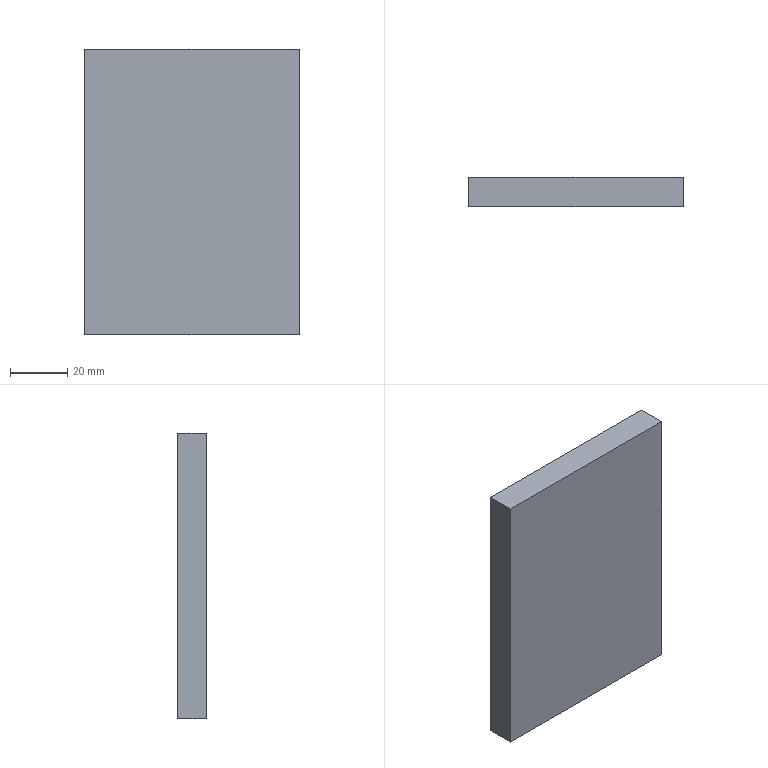Component | SolidWorks | TrolleyLeg-1_100X75X8-1 | 1 solid | 6 faces | box 75 x 10 x 100 mm | volume 75000 mm3 | plane 6 | material Plain Carbon Steel
STEP:
#1=COLOUR_RGB('',0.7922,0.8196,0.9333);
#2=FILL_AREA_STYLE_COLOUR('',#1);
#3=FILL_AREA_STYLE('',(#2));
#4=SURFACE_STYLE_FILL_AREA(#3);
#5=SURFACE_SIDE_STYLE('',(#4));
#6=SURFACE_STYLE_USAGE(.BOTH.,#5);
#7=PRESENTATION_STYLE_ASSIGNMENT((#6));
#8=CARTESIAN_POINT('',(-113.669,79.737,189.212));
#9=VERTEX_POINT('',#8);
#10=CARTESIAN_POINT('',(-113.669,79.737,185.275));
#11=VERTEX_POINT('',#10);
#12=CARTESIAN_POINT('',(-113.669,79.737,189.212));
#13=DIRECTION('',(0.,0.,-1.));
#14=VECTOR('',#13,39.37);
#15=LINE('',#12,#14);
#16=EDGE_CURVE('',#9,#11,#15,.T.);
#17=ORIENTED_EDGE('',*,*,#16,.F.);
#18=CARTESIAN_POINT('',(-113.669,80.131,189.212));
#19=VERTEX_POINT('',#18);
#20=CARTESIAN_POINT('',(-113.669,80.131,189.212));
#21=DIRECTION('',(0.,-1.,-0.));
#22=VECTOR('',#21,39.37);
#23=LINE('',#20,#22);
#24=EDGE_CURVE('',#19,#9,#23,.T.);
#25=ORIENTED_EDGE('',*,*,#24,.F.);
#26=CARTESIAN_POINT('',(-113.669,80.131,185.275));
#27=VERTEX_POINT('',#26);
#28=CARTESIAN_POINT('',(-113.669,80.131,189.212));
#29=DIRECTION('',(0.,0.,-1.));
#30=VECTOR('',#29,39.37);
#31=LINE('',#28,#30);
#32=EDGE_CURVE('',#19,#27,#31,.T.);
#33=ORIENTED_EDGE('',*,*,#32,.T.);
#34=CARTESIAN_POINT('',(-113.669,80.131,185.275));
#35=DIRECTION('',(0.,-1.,-0.));
#36=VECTOR('',#35,39.37);
#37=LINE('',#34,#36);
#38=EDGE_CURVE('',#27,#11,#37,.T.);
#39=ORIENTED_EDGE('',*,*,#38,.T.);
#40=EDGE_LOOP('',(#17,#25,#33,#39));
#41=FACE_OUTER_BOUND('',#40,.T.);
#42=CARTESIAN_POINT('',(-113.669,80.131,189.212));
#43=DIRECTION('',(-1.,0.,-0.));
#44=DIRECTION('',(0.,0.,-1.));
#45=AXIS2_PLACEMENT_3D('',#42,#43,#44);
#46=PLANE('',#45);
#47=ADVANCED_FACE('',(#41),#46,.T.);
#48=CARTESIAN_POINT('',(-110.717,79.737,189.212));
#49=VERTEX_POINT('',#48);
#50=CARTESIAN_POINT('',(-113.669,79.737,189.212));
#51=DIRECTION('',(-1.,0.,0.));
#52=VECTOR('',#51,39.37);
#53=LINE('',#50,#52);
#54=EDGE_CURVE('',#49,#9,#53,.T.);
#55=ORIENTED_EDGE('',*,*,#54,.F.);
#56=CARTESIAN_POINT('',(-110.717,80.131,189.212));
#57=VERTEX_POINT('',#56);
#58=CARTESIAN_POINT('',(-110.717,80.131,189.212));
#59=DIRECTION('',(0.,-1.,-0.));
#60=VECTOR('',#59,39.37);
#61=LINE('',#58,#60);
#62=EDGE_CURVE('',#57,#49,#61,.T.);
#63=ORIENTED_EDGE('',*,*,#62,.F.);
#64=CARTESIAN_POINT('',(-113.669,80.131,189.212));
#65=DIRECTION('',(-1.,0.,0.));
#66=VECTOR('',#65,39.37);
#67=LINE('',#64,#66);
#68=EDGE_CURVE('',#57,#19,#67,.T.);
#69=ORIENTED_EDGE('',*,*,#68,.T.);
#70=ORIENTED_EDGE('',*,*,#24,.T.);
#71=EDGE_LOOP('',(#55,#63,#69,#70));
#72=FACE_OUTER_BOUND('',#71,.T.);
#73=CARTESIAN_POINT('',(-113.669,80.131,189.212));
#74=DIRECTION('',(0.,-0.,1.));
#75=DIRECTION('',(-1.,0.,0.));
#76=AXIS2_PLACEMENT_3D('',#73,#74,#75);
#77=PLANE('',#76);
#78=ADVANCED_FACE('',(#72),#77,.T.);
#79=CARTESIAN_POINT('',(-110.717,79.737,185.275));
#80=VERTEX_POINT('',#79);
#81=CARTESIAN_POINT('',(-110.717,79.737,189.212));
#82=DIRECTION('',(-0.,-0.,1.));
#83=VECTOR('',#82,39.37);
#84=LINE('',#81,#83);
#85=EDGE_CURVE('',#80,#49,#84,.T.);
#86=ORIENTED_EDGE('',*,*,#85,.F.);
#87=CARTESIAN_POINT('',(-110.717,80.131,185.275));
#88=VERTEX_POINT('',#87);
#89=CARTESIAN_POINT('',(-110.717,80.131,185.275));
#90=DIRECTION('',(0.,-1.,-0.));
#91=VECTOR('',#90,39.37);
#92=LINE('',#89,#91);
#93=EDGE_CURVE('',#88,#80,#92,.T.);
#94=ORIENTED_EDGE('',*,*,#93,.F.);
#95=CARTESIAN_POINT('',(-110.717,80.131,189.212));
#96=DIRECTION('',(-0.,-0.,1.));
#97=VECTOR('',#96,39.37);
#98=LINE('',#95,#97);
#99=EDGE_CURVE('',#88,#57,#98,.T.);
#100=ORIENTED_EDGE('',*,*,#99,.T.);
#101=ORIENTED_EDGE('',*,*,#62,.T.);
#102=EDGE_LOOP('',(#86,#94,#100,#101));
#103=FACE_OUTER_BOUND('',#102,.T.);
#104=CARTESIAN_POINT('',(-110.717,80.131,189.212));
#105=DIRECTION('',(1.,-0.,0.));
#106=DIRECTION('',(-0.,-0.,1.));
#107=AXIS2_PLACEMENT_3D('',#104,#105,#106);
#108=PLANE('',#107);
#109=ADVANCED_FACE('',(#103),#108,.T.);
#110=CARTESIAN_POINT('',(-113.669,79.737,185.275));
#111=DIRECTION('',(1.,0.,0.));
#112=VECTOR('',#111,39.37);
#113=LINE('',#110,#112);
#114=EDGE_CURVE('',#11,#80,#113,.T.);
#115=ORIENTED_EDGE('',*,*,#114,.F.);
#116=ORIENTED_EDGE('',*,*,#38,.F.);
#117=CARTESIAN_POINT('',(-113.669,80.131,185.275));
#118=DIRECTION('',(1.,0.,0.));
#119=VECTOR('',#118,39.37);
#120=LINE('',#117,#119);
#121=EDGE_CURVE('',#27,#88,#120,.T.);
#122=ORIENTED_EDGE('',*,*,#121,.T.);
#123=ORIENTED_EDGE('',*,*,#93,.T.);
#124=EDGE_LOOP('',(#115,#116,#122,#123));
#125=FACE_OUTER_BOUND('',#124,.T.);
#126=CARTESIAN_POINT('',(-113.669,80.131,185.275));
#127=DIRECTION('',(0.,0.,-1.));
#128=DIRECTION('',(1.,0.,0.));
#129=AXIS2_PLACEMENT_3D('',#126,#127,#128);
#130=PLANE('',#129);
#131=ADVANCED_FACE('',(#125),#130,.T.);
#132=ORIENTED_EDGE('',*,*,#32,.F.);
#133=ORIENTED_EDGE('',*,*,#68,.F.);
#134=ORIENTED_EDGE('',*,*,#99,.F.);
#135=ORIENTED_EDGE('',*,*,#121,.F.);
#136=EDGE_LOOP('',(#132,#133,#134,#135));
#137=FACE_OUTER_BOUND('',#136,.T.);
#138=CARTESIAN_POINT('',(-113.669,80.131,189.212));
#139=DIRECTION('',(0.,-1.,-0.));
#140=DIRECTION('',(0.,0.,-1.));
#141=AXIS2_PLACEMENT_3D('',#138,#139,#140);
#142=PLANE('',#141);
#143=ADVANCED_FACE('',(#137),#142,.F.);
#144=ORIENTED_EDGE('',*,*,#16,.T.);
#145=ORIENTED_EDGE('',*,*,#114,.T.);
#146=ORIENTED_EDGE('',*,*,#85,.T.);
#147=ORIENTED_EDGE('',*,*,#54,.T.);
#148=EDGE_LOOP('',(#144,#145,#146,#147));
#149=FACE_OUTER_BOUND('',#148,.T.);
#150=CARTESIAN_POINT('',(-113.669,79.737,189.212));
#151=DIRECTION('',(0.,-1.,-0.));
#152=DIRECTION('',(0.,0.,-1.));
#153=AXIS2_PLACEMENT_3D('',#150,#151,#152);
#154=PLANE('',#153);
#155=ADVANCED_FACE('',(#149),#154,.T.);
#156=CLOSED_SHELL('',(#47,#78,#109,#131,#143,#155));
#157=MANIFOLD_SOLID_BREP('',#156);
#158=STYLED_ITEM('',(#7),#157);
#159=PRESENTATION_LAYER_ASSIGNMENT('','',(#158));
#160=(LENGTH_UNIT()NAMED_UNIT(*)SI_UNIT($,.METRE.));
#161=LENGTH_MEASURE_WITH_UNIT(LENGTH_MEASURE(0.0254),#160);
#162=DIMENSIONAL_EXPONENTS(1.,0.,0.,0.,0.,0.,0.);
#163=(CONVERSION_BASED_UNIT('',#161)LENGTH_UNIT()NAMED_UNIT(#162));
#164=UNCERTAINTY_MEASURE_WITH_UNIT(LENGTH_MEASURE(0.00001),#163,'','');
#165=(NAMED_UNIT(*)PLANE_ANGLE_UNIT()SI_UNIT($,.RADIAN.));
#166=(NAMED_UNIT(*)SI_UNIT($,.STERADIAN.)SOLID_ANGLE_UNIT());
#167=(GEOMETRIC_REPRESENTATION_CONTEXT(3)GLOBAL_UNCERTAINTY_ASSIGNED_CONTEXT((#164))GLOBAL_UNIT_ASSIGNED_CONTEXT((#163,#165,#166))REPRESENTATION_CONTEXT('',''));
#168=MECHANICAL_DESIGN_GEOMETRIC_PRESENTATION_REPRESENTATION('',(#158),#167);
#169=CARTESIAN_POINT('',(0.,0.,0.));
#170=DIRECTION('',(0.,0.,1.));
#171=DIRECTION('',(1.,0.,0.));
#172=AXIS2_PLACEMENT_3D('',#169,#170,#171);
#173=(LENGTH_UNIT()NAMED_UNIT(*)SI_UNIT($,.METRE.));
#174=LENGTH_MEASURE_WITH_UNIT(LENGTH_MEASURE(0.0254),#173);
#175=DIMENSIONAL_EXPONENTS(1.,0.,0.,0.,0.,0.,0.);
#176=(CONVERSION_BASED_UNIT('',#174)LENGTH_UNIT()NAMED_UNIT(#175));
#177=UNCERTAINTY_MEASURE_WITH_UNIT(LENGTH_MEASURE(0.00001),#176,'','');
#178=(NAMED_UNIT(*)PLANE_ANGLE_UNIT()SI_UNIT($,.RADIAN.));
#179=(NAMED_UNIT(*)SI_UNIT($,.STERADIAN.)SOLID_ANGLE_UNIT());
#180=(GEOMETRIC_REPRESENTATION_CONTEXT(3)GLOBAL_UNCERTAINTY_ASSIGNED_CONTEXT((#177))GLOBAL_UNIT_ASSIGNED_CONTEXT((#176,#178,#179))REPRESENTATION_CONTEXT('',''));
#181=ADVANCED_BREP_SHAPE_REPRESENTATION('',(#157,#172),#180);